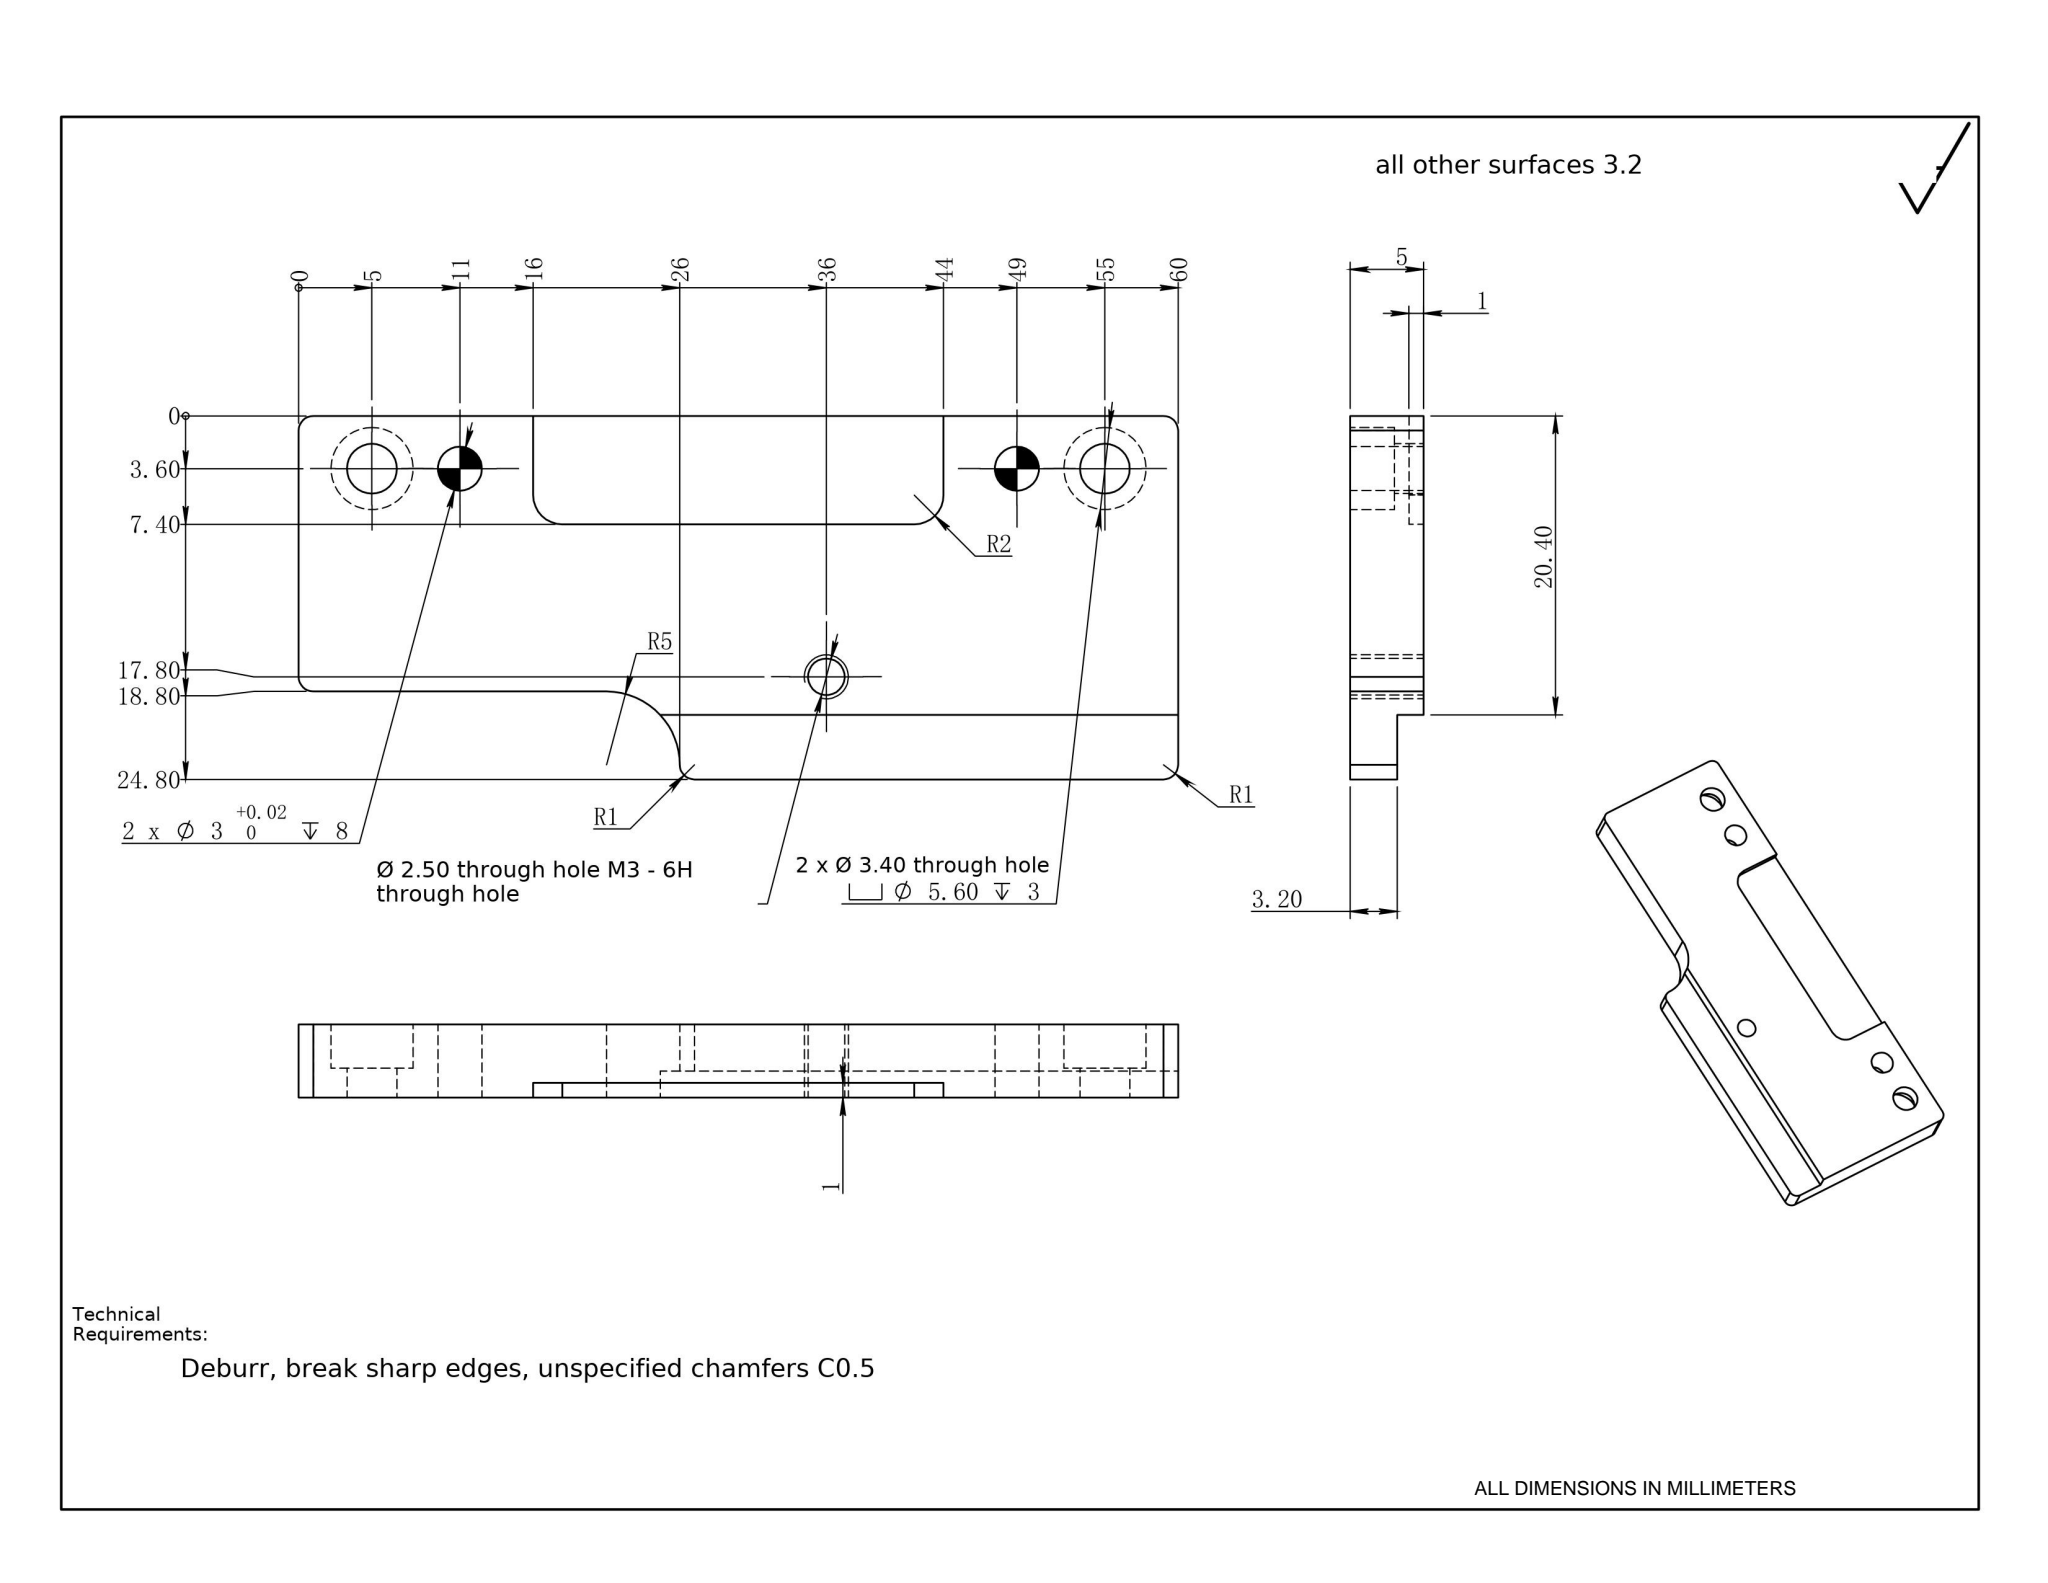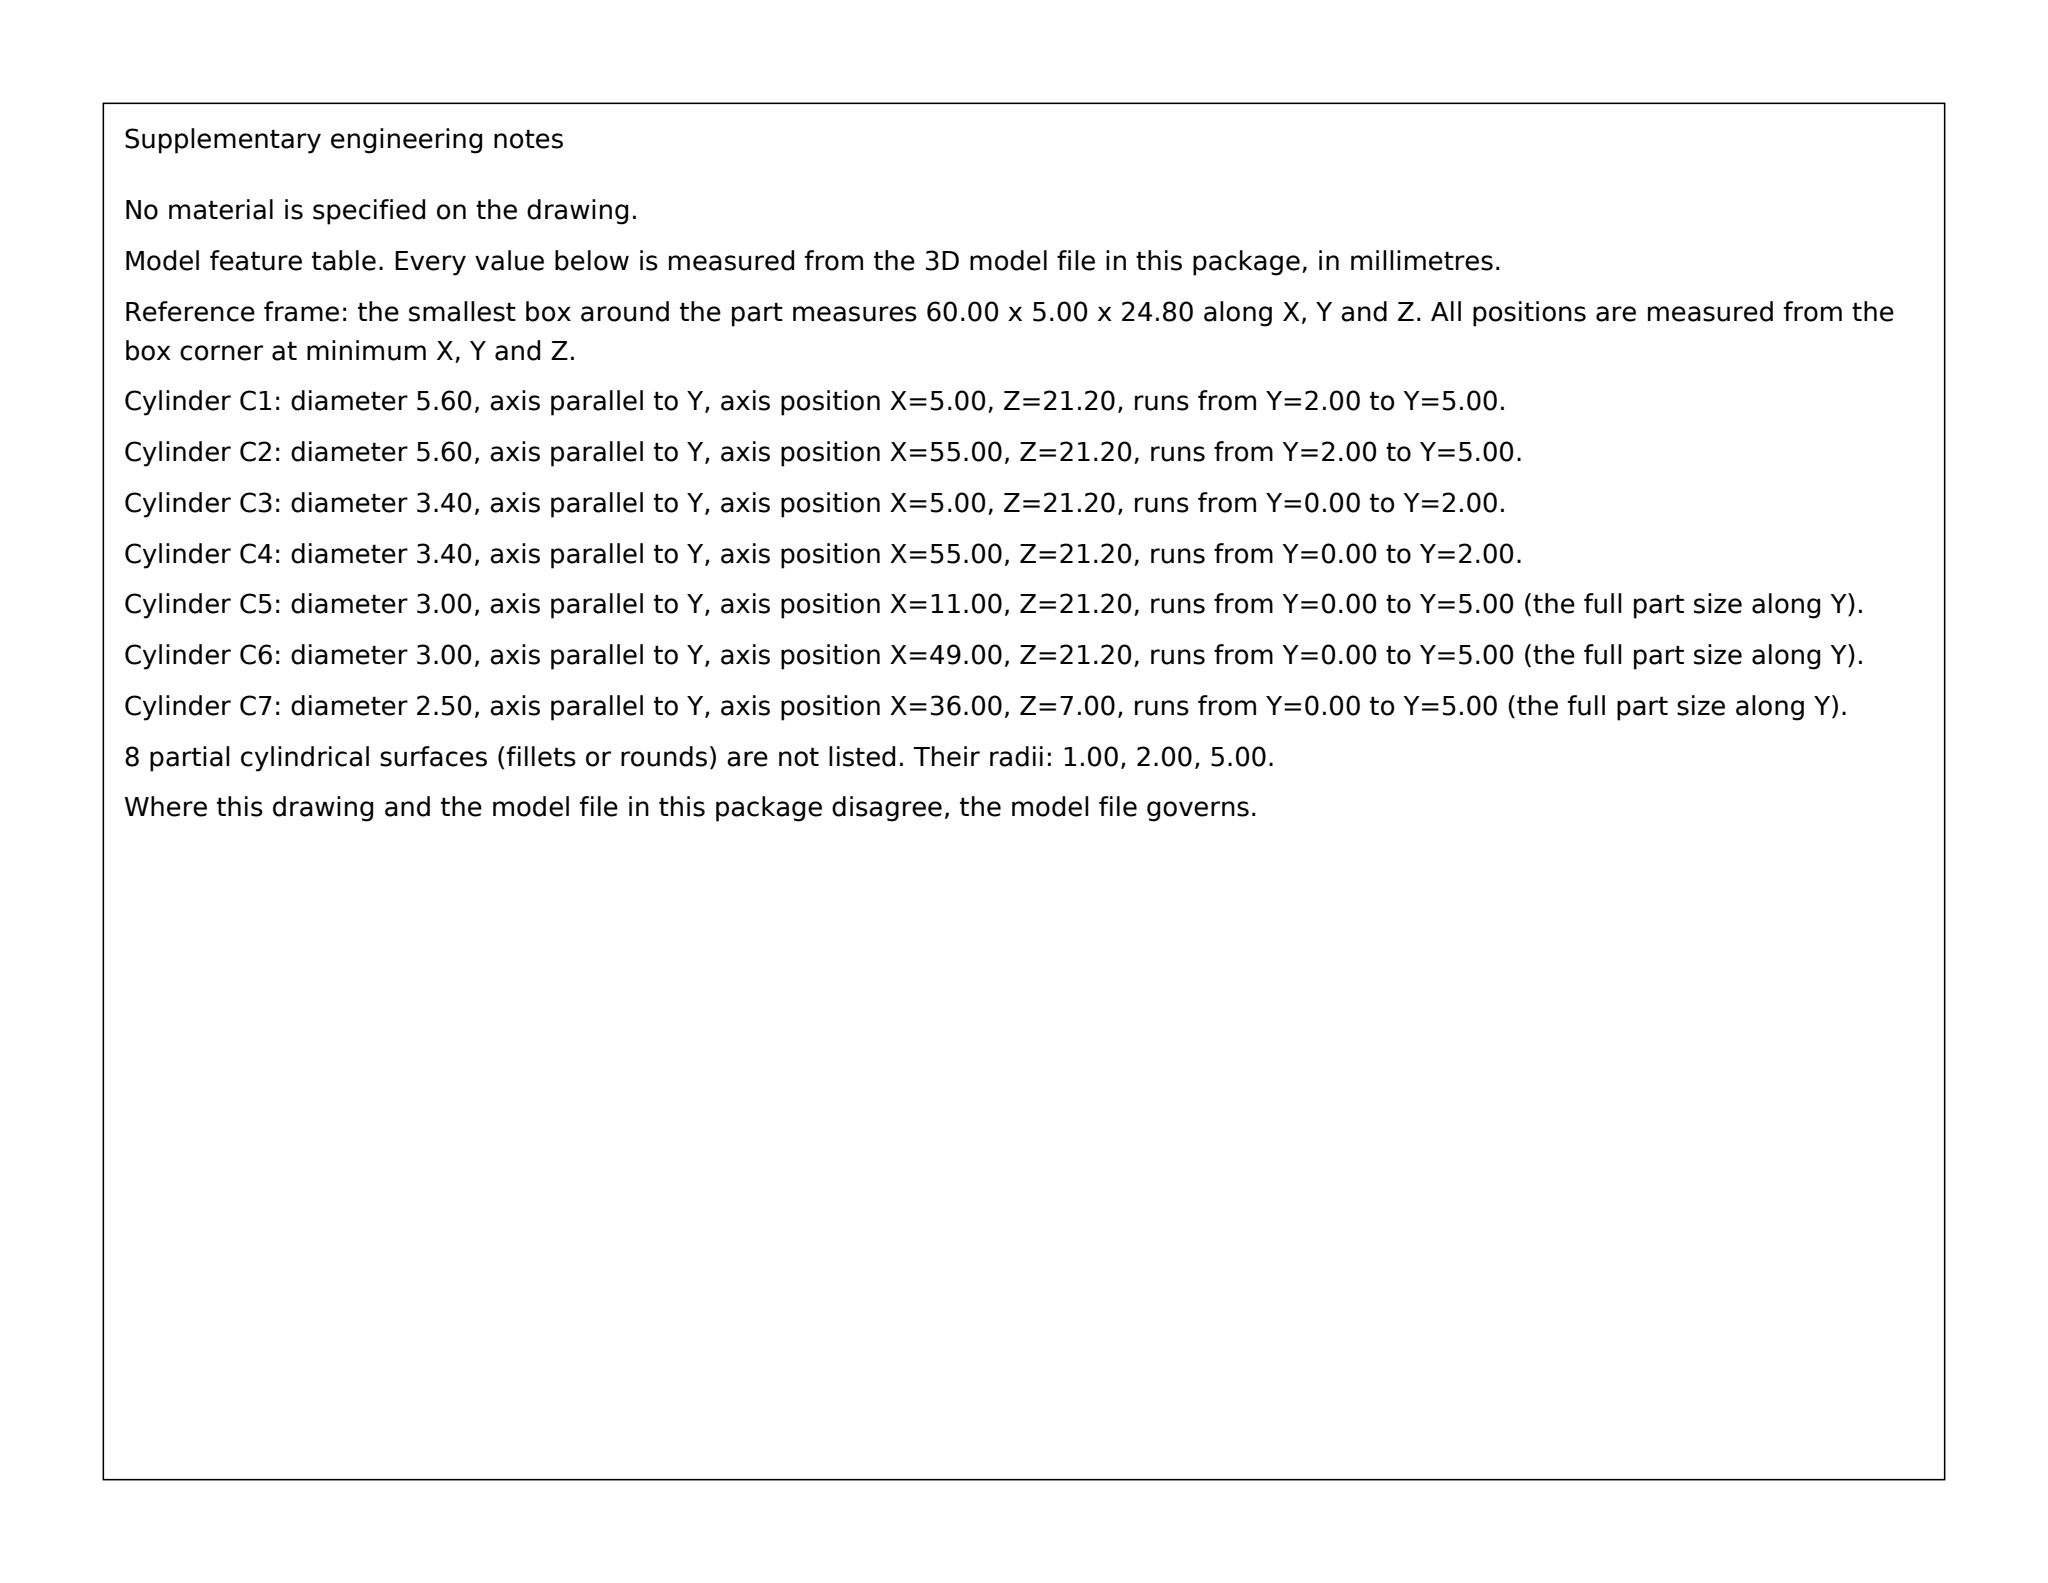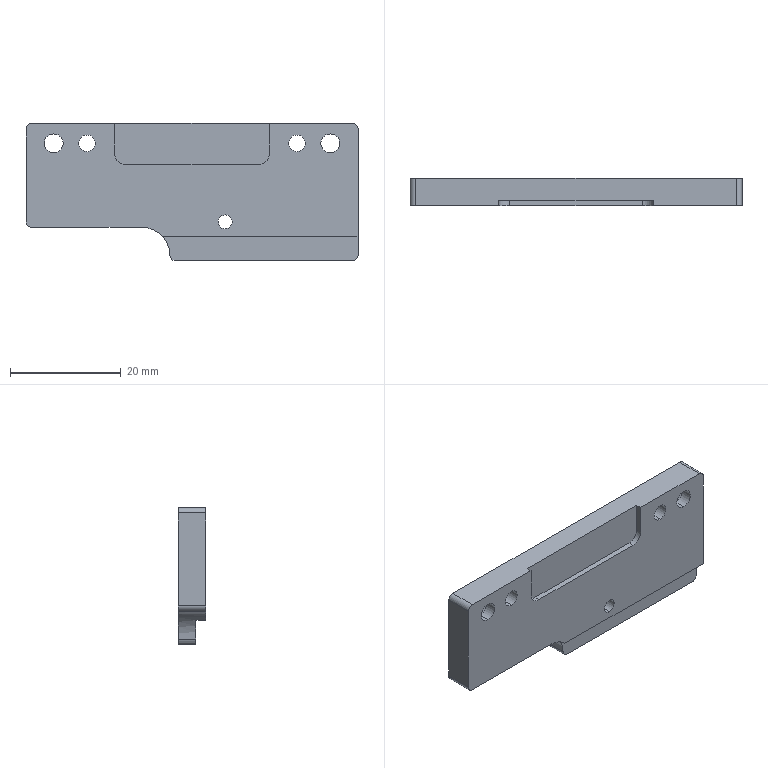Part | SolidWorks | mm | 1 solid | 37 faces | box 60 x 5 x 24.8 mm | volume 5926 mm3 | cylinder 22 | plane 15 | commonest cylinder face diameters 2 x5 3 x4 5.6 x4 3.4 x4 2.5 x2 4 x2 10 x1